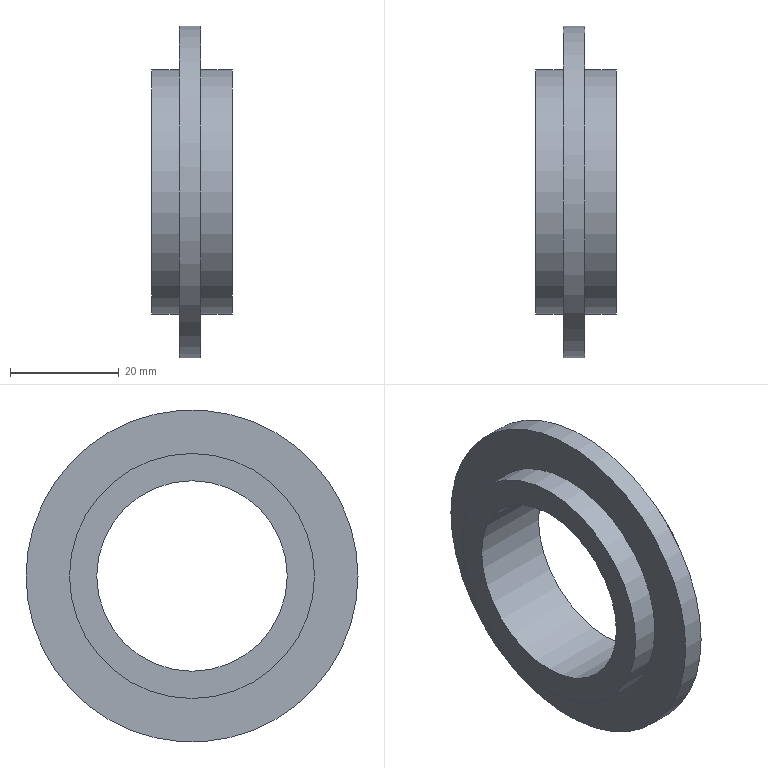Component | NX | DADANGYOUHUAN | 1 solid | 8 faces | box 14.75 x 61 x 61 mm | volume 14596 mm3 | cylinder 4 | plane 4 | commonest cylinder face diameters 45 x2 35 x1 61 x1
STEP:
#1=CARTESIAN_POINT('',(0.,0.,0.));
#2=DIRECTION('',(0.,0.,1.));
#3=DIRECTION('',(1.,0.,0.));
#4=AXIS2_PLACEMENT_3D('',#1,#2,#3);
#5=CARTESIAN_POINT('',(70.25,222.5,-88.));
#6=VERTEX_POINT('',#5);
#7=CARTESIAN_POINT('',(70.25,200.,-88.));
#8=DIRECTION('',(1.,0.,0.));
#9=DIRECTION('',(0.,1.,0.));
#10=AXIS2_PLACEMENT_3D('',#7,#8,#9);
#11=CIRCLE('',#10,22.5);
#12=CARTESIAN_POINT('',(85.,200.,-88.));
#13=DIRECTION('',(-1.,0.,0.));
#14=DIRECTION('',(0.,0.,1.));
#15=AXIS2_PLACEMENT_3D('',#12,#13,#14);
#16=CYLINDRICAL_SURFACE('',#15,22.5);
#17=CARTESIAN_POINT('',(7.854,14.75));
#18=DIRECTION('',(-1.,0.));
#19=VECTOR('',#18,1.);
#20=LINE('',#17,#19);
#21=(GEOMETRIC_REPRESENTATION_CONTEXT(2)PARAMETRIC_REPRESENTATION_CONTEXT()REPRESENTATION_CONTEXT('',''));
#22=DEFINITIONAL_REPRESENTATION('',(#20),#21);
#23=PCURVE('',#16,#22);
#24=CARTESIAN_POINT('',(70.25,200.,-88.));
#25=DIRECTION('',(1.,0.,0.));
#26=DIRECTION('',(0.,0.,-1.));
#27=AXIS2_PLACEMENT_3D('',#24,#25,#26);
#28=PLANE('',#27);
#29=CARTESIAN_POINT('',(0.,0.));
#30=DIRECTION('',(0.,1.));
#31=AXIS2_PLACEMENT_2D('',#29,#30);
#32=CIRCLE('',#31,22.5);
#33=(GEOMETRIC_REPRESENTATION_CONTEXT(2)PARAMETRIC_REPRESENTATION_CONTEXT()REPRESENTATION_CONTEXT('',''));
#34=DEFINITIONAL_REPRESENTATION('',(#32),#33);
#35=PCURVE('',#28,#34);
#36=SURFACE_CURVE('',#11,(#23,#35),.PCURVE_S1.);
#37=EDGE_CURVE('',#6,#6,#36,.T.);
#38=ORIENTED_EDGE('',*,*,#37,.T.);
#39=CARTESIAN_POINT('',(75.25,222.5,-88.));
#40=VERTEX_POINT('',#39);
#41=CARTESIAN_POINT('',(75.25,222.5,-88.));
#42=CARTESIAN_POINT('',(70.25,222.5,-88.));
#43=B_SPLINE_CURVE_WITH_KNOTS('',1,(#41,#42),.UNSPECIFIED.,.F.,.F.,(2,2),(9.75,14.75),.PIECEWISE_BEZIER_KNOTS.);
#44=CARTESIAN_POINT('',(1.571,0.));
#45=DIRECTION('',(0.,1.));
#46=VECTOR('',#45,1.);
#47=LINE('',#44,#46);
#48=(GEOMETRIC_REPRESENTATION_CONTEXT(2)PARAMETRIC_REPRESENTATION_CONTEXT()REPRESENTATION_CONTEXT('',''));
#49=DEFINITIONAL_REPRESENTATION('',(#47),#48);
#50=PCURVE('',#16,#49);
#51=CARTESIAN_POINT('',(7.854,0.));
#52=DIRECTION('',(0.,1.));
#53=VECTOR('',#52,1.);
#54=LINE('',#51,#53);
#55=(GEOMETRIC_REPRESENTATION_CONTEXT(2)PARAMETRIC_REPRESENTATION_CONTEXT()REPRESENTATION_CONTEXT('',''));
#56=DEFINITIONAL_REPRESENTATION('',(#54),#55);
#57=PCURVE('',#16,#56);
#58=SEAM_CURVE('',#43,(#50,#57),.PCURVE_S1.);
#59=EDGE_CURVE('',#40,#6,#58,.T.);
#60=ORIENTED_EDGE('',*,*,#59,.F.);
#61=CARTESIAN_POINT('',(75.25,200.,-110.5));
#62=VERTEX_POINT('',#61);
#63=CARTESIAN_POINT('',(75.25,200.,-88.));
#64=DIRECTION('',(1.,0.,0.));
#65=DIRECTION('',(0.,0.,-1.));
#66=AXIS2_PLACEMENT_3D('',#63,#64,#65);
#67=CIRCLE('',#66,22.5);
#68=CARTESIAN_POINT('',(3.142,9.75));
#69=DIRECTION('',(-1.,0.));
#70=VECTOR('',#69,1.);
#71=LINE('',#68,#70);
#72=(GEOMETRIC_REPRESENTATION_CONTEXT(2)PARAMETRIC_REPRESENTATION_CONTEXT()REPRESENTATION_CONTEXT('',''));
#73=DEFINITIONAL_REPRESENTATION('',(#71),#72);
#74=PCURVE('',#16,#73);
#75=CARTESIAN_POINT('',(75.25,200.,-88.));
#76=DIRECTION('',(1.,0.,0.));
#77=DIRECTION('',(0.,0.,-1.));
#78=AXIS2_PLACEMENT_3D('',#75,#76,#77);
#79=PLANE('',#78);
#80=CARTESIAN_POINT('',(0.,0.));
#81=DIRECTION('',(1.,0.));
#82=AXIS2_PLACEMENT_2D('',#80,#81);
#83=CIRCLE('',#82,22.5);
#84=(GEOMETRIC_REPRESENTATION_CONTEXT(2)PARAMETRIC_REPRESENTATION_CONTEXT()REPRESENTATION_CONTEXT('',''));
#85=DEFINITIONAL_REPRESENTATION('',(#83),#84);
#86=PCURVE('',#79,#85);
#87=SURFACE_CURVE('',#67,(#74,#86),.PCURVE_S1.);
#88=EDGE_CURVE('',#62,#40,#87,.T.);
#89=ORIENTED_EDGE('',*,*,#88,.F.);
#90=CARTESIAN_POINT('',(75.25,200.,-88.));
#91=DIRECTION('',(1.,0.,0.));
#92=DIRECTION('',(0.,0.,-1.));
#93=AXIS2_PLACEMENT_3D('',#90,#91,#92);
#94=CIRCLE('',#93,22.5);
#95=CARTESIAN_POINT('',(9.425,9.75));
#96=DIRECTION('',(-1.,0.));
#97=VECTOR('',#96,1.);
#98=LINE('',#95,#97);
#99=(GEOMETRIC_REPRESENTATION_CONTEXT(2)PARAMETRIC_REPRESENTATION_CONTEXT()REPRESENTATION_CONTEXT('',''));
#100=DEFINITIONAL_REPRESENTATION('',(#98),#99);
#101=PCURVE('',#16,#100);
#102=CARTESIAN_POINT('',(0.,0.));
#103=DIRECTION('',(1.,0.));
#104=AXIS2_PLACEMENT_2D('',#102,#103);
#105=CIRCLE('',#104,22.5);
#106=(GEOMETRIC_REPRESENTATION_CONTEXT(2)PARAMETRIC_REPRESENTATION_CONTEXT()REPRESENTATION_CONTEXT('',''));
#107=DEFINITIONAL_REPRESENTATION('',(#105),#106);
#108=PCURVE('',#79,#107);
#109=SURFACE_CURVE('',#94,(#101,#108),.PCURVE_S1.);
#110=EDGE_CURVE('',#40,#62,#109,.T.);
#111=ORIENTED_EDGE('',*,*,#110,.F.);
#112=ORIENTED_EDGE('',*,*,#59,.T.);
#113=EDGE_LOOP('',(#38,#60,#89,#111,#112));
#114=FACE_BOUND('',#113,.T.);
#115=ADVANCED_FACE('',(#114),#16,.T.);
#116=CARTESIAN_POINT('',(79.25,222.5,-88.));
#117=VERTEX_POINT('',#116);
#118=CARTESIAN_POINT('',(79.25,200.,-88.));
#119=DIRECTION('',(1.,0.,0.));
#120=DIRECTION('',(0.,1.,0.));
#121=AXIS2_PLACEMENT_3D('',#118,#119,#120);
#122=CIRCLE('',#121,22.5);
#123=CARTESIAN_POINT('',(85.,200.,-88.));
#124=DIRECTION('',(-1.,0.,0.));
#125=DIRECTION('',(0.,0.,1.));
#126=AXIS2_PLACEMENT_3D('',#123,#124,#125);
#127=CYLINDRICAL_SURFACE('',#126,22.5);
#128=CARTESIAN_POINT('',(7.854,5.75));
#129=DIRECTION('',(-1.,0.));
#130=VECTOR('',#129,1.);
#131=LINE('',#128,#130);
#132=(GEOMETRIC_REPRESENTATION_CONTEXT(2)PARAMETRIC_REPRESENTATION_CONTEXT()REPRESENTATION_CONTEXT('',''));
#133=DEFINITIONAL_REPRESENTATION('',(#131),#132);
#134=PCURVE('',#127,#133);
#135=CARTESIAN_POINT('',(79.25,200.,-88.));
#136=DIRECTION('',(1.,0.,0.));
#137=DIRECTION('',(0.,0.,-1.));
#138=AXIS2_PLACEMENT_3D('',#135,#136,#137);
#139=PLANE('',#138);
#140=CARTESIAN_POINT('',(0.,0.));
#141=DIRECTION('',(0.,1.));
#142=AXIS2_PLACEMENT_2D('',#140,#141);
#143=CIRCLE('',#142,22.5);
#144=(GEOMETRIC_REPRESENTATION_CONTEXT(2)PARAMETRIC_REPRESENTATION_CONTEXT()REPRESENTATION_CONTEXT('',''));
#145=DEFINITIONAL_REPRESENTATION('',(#143),#144);
#146=PCURVE('',#139,#145);
#147=SURFACE_CURVE('',#122,(#134,#146),.PCURVE_S1.);
#148=EDGE_CURVE('',#117,#117,#147,.T.);
#149=ORIENTED_EDGE('',*,*,#148,.T.);
#150=CARTESIAN_POINT('',(85.,222.5,-88.));
#151=VERTEX_POINT('',#150);
#152=CARTESIAN_POINT('',(85.,222.5,-88.));
#153=CARTESIAN_POINT('',(79.25,222.5,-88.));
#154=B_SPLINE_CURVE_WITH_KNOTS('',1,(#152,#153),.UNSPECIFIED.,.F.,.F.,(2,2),(0.,5.75),.PIECEWISE_BEZIER_KNOTS.);
#155=CARTESIAN_POINT('',(1.571,0.));
#156=DIRECTION('',(0.,1.));
#157=VECTOR('',#156,1.);
#158=LINE('',#155,#157);
#159=(GEOMETRIC_REPRESENTATION_CONTEXT(2)PARAMETRIC_REPRESENTATION_CONTEXT()REPRESENTATION_CONTEXT('',''));
#160=DEFINITIONAL_REPRESENTATION('',(#158),#159);
#161=PCURVE('',#127,#160);
#162=CARTESIAN_POINT('',(7.854,0.));
#163=DIRECTION('',(0.,1.));
#164=VECTOR('',#163,1.);
#165=LINE('',#162,#164);
#166=(GEOMETRIC_REPRESENTATION_CONTEXT(2)PARAMETRIC_REPRESENTATION_CONTEXT()REPRESENTATION_CONTEXT('',''));
#167=DEFINITIONAL_REPRESENTATION('',(#165),#166);
#168=PCURVE('',#127,#167);
#169=SEAM_CURVE('',#154,(#161,#168),.PCURVE_S1.);
#170=EDGE_CURVE('',#151,#117,#169,.T.);
#171=ORIENTED_EDGE('',*,*,#170,.F.);
#172=CARTESIAN_POINT('',(85.,200.,-88.));
#173=DIRECTION('',(1.,0.,0.));
#174=DIRECTION('',(0.,1.,0.));
#175=AXIS2_PLACEMENT_3D('',#172,#173,#174);
#176=CIRCLE('',#175,22.5);
#177=CARTESIAN_POINT('',(7.854,0.));
#178=DIRECTION('',(-1.,0.));
#179=VECTOR('',#178,1.);
#180=LINE('',#177,#179);
#181=(GEOMETRIC_REPRESENTATION_CONTEXT(2)PARAMETRIC_REPRESENTATION_CONTEXT()REPRESENTATION_CONTEXT('',''));
#182=DEFINITIONAL_REPRESENTATION('',(#180),#181);
#183=PCURVE('',#127,#182);
#184=CARTESIAN_POINT('',(85.,200.,-88.));
#185=DIRECTION('',(1.,0.,0.));
#186=DIRECTION('',(0.,0.,-1.));
#187=AXIS2_PLACEMENT_3D('',#184,#185,#186);
#188=PLANE('',#187);
#189=CARTESIAN_POINT('',(0.,0.));
#190=DIRECTION('',(0.,1.));
#191=AXIS2_PLACEMENT_2D('',#189,#190);
#192=CIRCLE('',#191,22.5);
#193=(GEOMETRIC_REPRESENTATION_CONTEXT(2)PARAMETRIC_REPRESENTATION_CONTEXT()REPRESENTATION_CONTEXT('',''));
#194=DEFINITIONAL_REPRESENTATION('',(#192),#193);
#195=PCURVE('',#188,#194);
#196=SURFACE_CURVE('',#176,(#183,#195),.PCURVE_S1.);
#197=EDGE_CURVE('',#151,#151,#196,.T.);
#198=ORIENTED_EDGE('',*,*,#197,.F.);
#199=ORIENTED_EDGE('',*,*,#170,.T.);
#200=EDGE_LOOP('',(#149,#171,#198,#199));
#201=FACE_BOUND('',#200,.T.);
#202=ADVANCED_FACE('',(#201),#127,.T.);
#203=CARTESIAN_POINT('',(85.,217.5,-88.));
#204=VERTEX_POINT('',#203);
#205=CARTESIAN_POINT('',(85.,200.,-88.));
#206=DIRECTION('',(1.,0.,0.));
#207=DIRECTION('',(0.,1.,0.));
#208=AXIS2_PLACEMENT_3D('',#205,#206,#207);
#209=CIRCLE('',#208,17.5);
#210=CARTESIAN_POINT('',(85.,200.,-88.));
#211=DIRECTION('',(-1.,0.,0.));
#212=DIRECTION('',(0.,0.,1.));
#213=AXIS2_PLACEMENT_3D('',#210,#211,#212);
#214=CYLINDRICAL_SURFACE('',#213,17.5);
#215=CARTESIAN_POINT('',(7.854,0.));
#216=DIRECTION('',(-1.,0.));
#217=VECTOR('',#216,1.);
#218=LINE('',#215,#217);
#219=(GEOMETRIC_REPRESENTATION_CONTEXT(2)PARAMETRIC_REPRESENTATION_CONTEXT()REPRESENTATION_CONTEXT('',''));
#220=DEFINITIONAL_REPRESENTATION('',(#218),#219);
#221=PCURVE('',#214,#220);
#222=CARTESIAN_POINT('',(0.,0.));
#223=DIRECTION('',(0.,1.));
#224=AXIS2_PLACEMENT_2D('',#222,#223);
#225=CIRCLE('',#224,17.5);
#226=(GEOMETRIC_REPRESENTATION_CONTEXT(2)PARAMETRIC_REPRESENTATION_CONTEXT()REPRESENTATION_CONTEXT('',''));
#227=DEFINITIONAL_REPRESENTATION('',(#225),#226);
#228=PCURVE('',#188,#227);
#229=SURFACE_CURVE('',#209,(#221,#228),.PCURVE_S1.);
#230=EDGE_CURVE('',#204,#204,#229,.T.);
#231=ORIENTED_EDGE('',*,*,#230,.F.);
#232=CARTESIAN_POINT('',(70.25,217.5,-88.));
#233=VERTEX_POINT('',#232);
#234=CARTESIAN_POINT('',(85.,217.5,-88.));
#235=CARTESIAN_POINT('',(70.25,217.5,-88.));
#236=B_SPLINE_CURVE_WITH_KNOTS('',1,(#234,#235),.UNSPECIFIED.,.F.,.F.,(2,2),(0.,14.75),.PIECEWISE_BEZIER_KNOTS.);
#237=CARTESIAN_POINT('',(7.854,0.));
#238=DIRECTION('',(0.,1.));
#239=VECTOR('',#238,1.);
#240=LINE('',#237,#239);
#241=(GEOMETRIC_REPRESENTATION_CONTEXT(2)PARAMETRIC_REPRESENTATION_CONTEXT()REPRESENTATION_CONTEXT('',''));
#242=DEFINITIONAL_REPRESENTATION('',(#240),#241);
#243=PCURVE('',#214,#242);
#244=CARTESIAN_POINT('',(1.571,0.));
#245=DIRECTION('',(0.,1.));
#246=VECTOR('',#245,1.);
#247=LINE('',#244,#246);
#248=(GEOMETRIC_REPRESENTATION_CONTEXT(2)PARAMETRIC_REPRESENTATION_CONTEXT()REPRESENTATION_CONTEXT('',''));
#249=DEFINITIONAL_REPRESENTATION('',(#247),#248);
#250=PCURVE('',#214,#249);
#251=SEAM_CURVE('',#236,(#243,#250),.PCURVE_S1.);
#252=EDGE_CURVE('',#204,#233,#251,.T.);
#253=ORIENTED_EDGE('',*,*,#252,.T.);
#254=CARTESIAN_POINT('',(70.25,200.,-88.));
#255=DIRECTION('',(1.,0.,0.));
#256=DIRECTION('',(0.,1.,0.));
#257=AXIS2_PLACEMENT_3D('',#254,#255,#256);
#258=CIRCLE('',#257,17.5);
#259=CARTESIAN_POINT('',(7.854,14.75));
#260=DIRECTION('',(-1.,0.));
#261=VECTOR('',#260,1.);
#262=LINE('',#259,#261);
#263=(GEOMETRIC_REPRESENTATION_CONTEXT(2)PARAMETRIC_REPRESENTATION_CONTEXT()REPRESENTATION_CONTEXT('',''));
#264=DEFINITIONAL_REPRESENTATION('',(#262),#263);
#265=PCURVE('',#214,#264);
#266=CARTESIAN_POINT('',(0.,0.));
#267=DIRECTION('',(0.,1.));
#268=AXIS2_PLACEMENT_2D('',#266,#267);
#269=CIRCLE('',#268,17.5);
#270=(GEOMETRIC_REPRESENTATION_CONTEXT(2)PARAMETRIC_REPRESENTATION_CONTEXT()REPRESENTATION_CONTEXT('',''));
#271=DEFINITIONAL_REPRESENTATION('',(#269),#270);
#272=PCURVE('',#28,#271);
#273=SURFACE_CURVE('',#258,(#265,#272),.PCURVE_S1.);
#274=EDGE_CURVE('',#233,#233,#273,.T.);
#275=ORIENTED_EDGE('',*,*,#274,.T.);
#276=ORIENTED_EDGE('',*,*,#252,.F.);
#277=EDGE_LOOP('',(#231,#253,#275,#276));
#278=FACE_BOUND('',#277,.F.);
#279=ADVANCED_FACE('',(#278),#214,.F.);
#280=ORIENTED_EDGE('',*,*,#197,.T.);
#281=EDGE_LOOP('',(#280));
#282=FACE_BOUND('',#281,.T.);
#283=ORIENTED_EDGE('',*,*,#230,.F.);
#284=EDGE_LOOP('',(#283));
#285=FACE_BOUND('',#284,.T.);
#286=ADVANCED_FACE('',(#282,#285),#188,.T.);
#287=ORIENTED_EDGE('',*,*,#37,.F.);
#288=EDGE_LOOP('',(#287));
#289=FACE_BOUND('',#288,.T.);
#290=ORIENTED_EDGE('',*,*,#274,.T.);
#291=EDGE_LOOP('',(#290));
#292=FACE_BOUND('',#291,.T.);
#293=ADVANCED_FACE('',(#289,#292),#28,.F.);
#294=CARTESIAN_POINT('',(79.25,230.5,-88.));
#295=VERTEX_POINT('',#294);
#296=CARTESIAN_POINT('',(79.25,200.,-88.));
#297=DIRECTION('',(1.,0.,0.));
#298=DIRECTION('',(0.,1.,0.));
#299=AXIS2_PLACEMENT_3D('',#296,#297,#298);
#300=CIRCLE('',#299,30.5);
#301=CARTESIAN_POINT('',(79.25,200.,-88.));
#302=DIRECTION('',(-1.,0.,0.));
#303=DIRECTION('',(0.,0.,1.));
#304=AXIS2_PLACEMENT_3D('',#301,#302,#303);
#305=CYLINDRICAL_SURFACE('',#304,30.5);
#306=CARTESIAN_POINT('',(7.854,0.));
#307=DIRECTION('',(-1.,0.));
#308=VECTOR('',#307,1.);
#309=LINE('',#306,#308);
#310=(GEOMETRIC_REPRESENTATION_CONTEXT(2)PARAMETRIC_REPRESENTATION_CONTEXT()REPRESENTATION_CONTEXT('',''));
#311=DEFINITIONAL_REPRESENTATION('',(#309),#310);
#312=PCURVE('',#305,#311);
#313=CARTESIAN_POINT('',(0.,0.));
#314=DIRECTION('',(0.,1.));
#315=AXIS2_PLACEMENT_2D('',#313,#314);
#316=CIRCLE('',#315,30.5);
#317=(GEOMETRIC_REPRESENTATION_CONTEXT(2)PARAMETRIC_REPRESENTATION_CONTEXT()REPRESENTATION_CONTEXT('',''));
#318=DEFINITIONAL_REPRESENTATION('',(#316),#317);
#319=PCURVE('',#139,#318);
#320=SURFACE_CURVE('',#300,(#312,#319),.PCURVE_S1.);
#321=EDGE_CURVE('',#295,#295,#320,.T.);
#322=ORIENTED_EDGE('',*,*,#321,.F.);
#323=CARTESIAN_POINT('',(75.25,230.5,-88.));
#324=VERTEX_POINT('',#323);
#325=CARTESIAN_POINT('',(79.25,230.5,-88.));
#326=CARTESIAN_POINT('',(75.25,230.5,-88.));
#327=B_SPLINE_CURVE_WITH_KNOTS('',1,(#325,#326),.UNSPECIFIED.,.F.,.F.,(2,2),(0.,4.),.PIECEWISE_BEZIER_KNOTS.);
#328=CARTESIAN_POINT('',(7.854,0.));
#329=DIRECTION('',(0.,1.));
#330=VECTOR('',#329,1.);
#331=LINE('',#328,#330);
#332=(GEOMETRIC_REPRESENTATION_CONTEXT(2)PARAMETRIC_REPRESENTATION_CONTEXT()REPRESENTATION_CONTEXT('',''));
#333=DEFINITIONAL_REPRESENTATION('',(#331),#332);
#334=PCURVE('',#305,#333);
#335=CARTESIAN_POINT('',(1.571,0.));
#336=DIRECTION('',(0.,1.));
#337=VECTOR('',#336,1.);
#338=LINE('',#335,#337);
#339=(GEOMETRIC_REPRESENTATION_CONTEXT(2)PARAMETRIC_REPRESENTATION_CONTEXT()REPRESENTATION_CONTEXT('',''));
#340=DEFINITIONAL_REPRESENTATION('',(#338),#339);
#341=PCURVE('',#305,#340);
#342=SEAM_CURVE('',#327,(#334,#341),.PCURVE_S1.);
#343=EDGE_CURVE('',#295,#324,#342,.T.);
#344=ORIENTED_EDGE('',*,*,#343,.T.);
#345=CARTESIAN_POINT('',(75.25,200.,-88.));
#346=DIRECTION('',(1.,0.,0.));
#347=DIRECTION('',(0.,1.,0.));
#348=AXIS2_PLACEMENT_3D('',#345,#346,#347);
#349=CIRCLE('',#348,30.5);
#350=CARTESIAN_POINT('',(7.854,4.));
#351=DIRECTION('',(-1.,0.));
#352=VECTOR('',#351,1.);
#353=LINE('',#350,#352);
#354=(GEOMETRIC_REPRESENTATION_CONTEXT(2)PARAMETRIC_REPRESENTATION_CONTEXT()REPRESENTATION_CONTEXT('',''));
#355=DEFINITIONAL_REPRESENTATION('',(#353),#354);
#356=PCURVE('',#305,#355);
#357=CARTESIAN_POINT('',(0.,0.));
#358=DIRECTION('',(0.,1.));
#359=AXIS2_PLACEMENT_2D('',#357,#358);
#360=CIRCLE('',#359,30.5);
#361=(GEOMETRIC_REPRESENTATION_CONTEXT(2)PARAMETRIC_REPRESENTATION_CONTEXT()REPRESENTATION_CONTEXT('',''));
#362=DEFINITIONAL_REPRESENTATION('',(#360),#361);
#363=PCURVE('',#79,#362);
#364=SURFACE_CURVE('',#349,(#356,#363),.PCURVE_S1.);
#365=EDGE_CURVE('',#324,#324,#364,.T.);
#366=ORIENTED_EDGE('',*,*,#365,.T.);
#367=ORIENTED_EDGE('',*,*,#343,.F.);
#368=EDGE_LOOP('',(#322,#344,#366,#367));
#369=FACE_BOUND('',#368,.T.);
#370=ADVANCED_FACE('',(#369),#305,.T.);
#371=ORIENTED_EDGE('',*,*,#321,.T.);
#372=EDGE_LOOP('',(#371));
#373=FACE_BOUND('',#372,.T.);
#374=ORIENTED_EDGE('',*,*,#148,.F.);
#375=EDGE_LOOP('',(#374));
#376=FACE_BOUND('',#375,.T.);
#377=ADVANCED_FACE('',(#373,#376),#139,.T.);
#378=ORIENTED_EDGE('',*,*,#365,.F.);
#379=EDGE_LOOP('',(#378));
#380=FACE_BOUND('',#379,.T.);
#381=ORIENTED_EDGE('',*,*,#88,.T.);
#382=ORIENTED_EDGE('',*,*,#110,.T.);
#383=EDGE_LOOP('',(#381,#382));
#384=FACE_BOUND('',#383,.T.);
#385=ADVANCED_FACE('',(#380,#384),#79,.F.);
#386=CLOSED_SHELL('',(#115,#202,#279,#286,#293,#370,#377,#385));
#387=MANIFOLD_SOLID_BREP('',#386);
#388=(LENGTH_UNIT()NAMED_UNIT(*)SI_UNIT(.MILLI.,.METRE.));
#389=UNCERTAINTY_MEASURE_WITH_UNIT(LENGTH_MEASURE(0.000005),#388,'','');
#390=(NAMED_UNIT(*)PLANE_ANGLE_UNIT()SI_UNIT($,.RADIAN.));
#391=(NAMED_UNIT(*)SI_UNIT($,.STERADIAN.)SOLID_ANGLE_UNIT());
#392=(GEOMETRIC_REPRESENTATION_CONTEXT(3)GLOBAL_UNCERTAINTY_ASSIGNED_CONTEXT((#389))GLOBAL_UNIT_ASSIGNED_CONTEXT((#388,#390,#391))REPRESENTATION_CONTEXT('',''));
#393=ADVANCED_BREP_SHAPE_REPRESENTATION('',(#4,#387),#392);